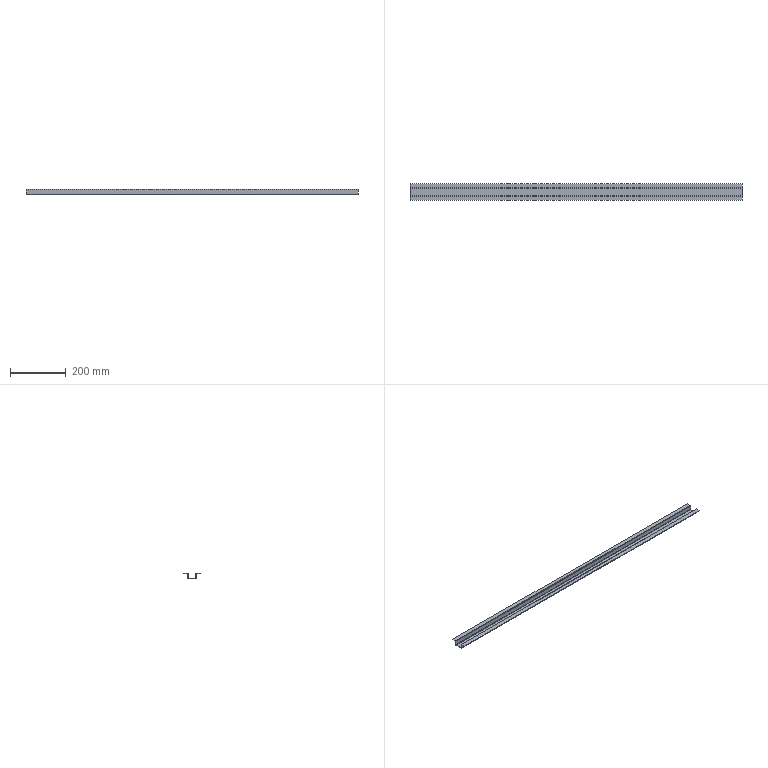Component | SolidWorks | TopPlate-1_TopPanelStiffener-2 | 1 solid | 38 faces | box 1196 x 60 x 18.4 mm | volume 88788 mm3 | plane 30 | cylinder 8 | commonest cylinder face diameters 3.6 x4 2 x4 | material 304
STEP:
#1=COLOUR_RGB('',0.7922,0.8196,0.9333);
#2=FILL_AREA_STYLE_COLOUR('',#1);
#3=FILL_AREA_STYLE('',(#2));
#4=SURFACE_STYLE_FILL_AREA(#3);
#5=SURFACE_SIDE_STYLE('',(#4));
#6=SURFACE_STYLE_USAGE(.BOTH.,#5);
#7=PRESENTATION_STYLE_ASSIGNMENT((#6));
#8=CARTESIAN_POINT('',(-25.908,6.088,79.152));
#9=VERTEX_POINT('',#8);
#10=CARTESIAN_POINT('',(-25.908,6.119,79.152));
#11=VERTEX_POINT('',#10);
#12=CARTESIAN_POINT('',(-25.908,6.088,79.152));
#13=DIRECTION('',(0.,1.,0.));
#14=VECTOR('',#13,39.37);
#15=LINE('',#12,#14);
#16=EDGE_CURVE('',#9,#11,#15,.T.);
#17=ORIENTED_EDGE('',*,*,#16,.F.);
#18=CARTESIAN_POINT('',(-25.908,6.048,79.191));
#19=VERTEX_POINT('',#18);
#20=CARTESIAN_POINT('',(-25.908,6.048,79.152));
#21=DIRECTION('',(1.,-0.,0.));
#22=DIRECTION('',(0.,0.,-1.));
#23=AXIS2_PLACEMENT_3D('',#20,#21,#22);
#24=CIRCLE('',#23,0.03937);
#25=EDGE_CURVE('',#9,#19,#24,.T.);
#26=ORIENTED_EDGE('',*,*,#25,.T.);
#27=CARTESIAN_POINT('',(-25.908,6.048,79.222));
#28=VERTEX_POINT('',#27);
#29=CARTESIAN_POINT('',(-25.908,6.048,79.222));
#30=DIRECTION('',(0.,0.,-1.));
#31=VECTOR('',#30,39.37);
#32=LINE('',#29,#31);
#33=EDGE_CURVE('',#28,#19,#32,.T.);
#34=ORIENTED_EDGE('',*,*,#33,.F.);
#35=CARTESIAN_POINT('',(-25.908,6.048,79.152));
#36=DIRECTION('',(1.,-0.,0.));
#37=DIRECTION('',(0.,1.,0.));
#38=AXIS2_PLACEMENT_3D('',#35,#36,#37);
#39=CIRCLE('',#38,0.07087);
#40=EDGE_CURVE('',#11,#28,#39,.T.);
#41=ORIENTED_EDGE('',*,*,#40,.F.);
#42=EDGE_LOOP('',(#17,#26,#34,#41));
#43=FACE_OUTER_BOUND('',#42,.T.);
#44=CARTESIAN_POINT('',(-25.908,6.088,79.152));
#45=DIRECTION('',(-1.,0.,-0.));
#46=DIRECTION('',(-0.,-0.,1.));
#47=AXIS2_PLACEMENT_3D('',#44,#45,#46);
#48=PLANE('',#47);
#49=ADVANCED_FACE('',(#43),#48,.T.);
#50=CARTESIAN_POINT('',(-25.908,6.088,78.569));
#51=VERTEX_POINT('',#50);
#52=CARTESIAN_POINT('',(-25.908,6.088,79.191));
#53=DIRECTION('',(-0.,-0.,1.));
#54=VECTOR('',#53,39.37);
#55=LINE('',#52,#54);
#56=EDGE_CURVE('',#51,#9,#55,.T.);
#57=ORIENTED_EDGE('',*,*,#56,.T.);
#58=ORIENTED_EDGE('',*,*,#16,.T.);
#59=CARTESIAN_POINT('',(-25.908,6.119,78.569));
#60=VERTEX_POINT('',#59);
#61=CARTESIAN_POINT('',(-25.908,6.119,79.191));
#62=DIRECTION('',(-0.,-0.,1.));
#63=VECTOR('',#62,39.37);
#64=LINE('',#61,#63);
#65=EDGE_CURVE('',#60,#11,#64,.T.);
#66=ORIENTED_EDGE('',*,*,#65,.F.);
#67=CARTESIAN_POINT('',(-25.908,6.119,78.569));
#68=DIRECTION('',(-0.,-1.,-0.));
#69=VECTOR('',#68,39.37);
#70=LINE('',#67,#69);
#71=EDGE_CURVE('',#60,#51,#70,.T.);
#72=ORIENTED_EDGE('',*,*,#71,.T.);
#73=EDGE_LOOP('',(#57,#58,#66,#72));
#74=FACE_OUTER_BOUND('',#73,.T.);
#75=CARTESIAN_POINT('',(-25.908,6.048,79.222));
#76=DIRECTION('',(-1.,0.,-0.));
#77=DIRECTION('',(-0.,-0.,1.));
#78=AXIS2_PLACEMENT_3D('',#75,#76,#77);
#79=PLANE('',#78);
#80=ADVANCED_FACE('',(#74),#79,.T.);
#81=CARTESIAN_POINT('',(21.178,6.048,79.191));
#82=VERTEX_POINT('',#81);
#83=CARTESIAN_POINT('',(21.178,6.048,79.222));
#84=VERTEX_POINT('',#83);
#85=CARTESIAN_POINT('',(21.178,6.048,79.191));
#86=DIRECTION('',(-0.,-0.,1.));
#87=VECTOR('',#86,39.37);
#88=LINE('',#85,#87);
#89=EDGE_CURVE('',#82,#84,#88,.T.);
#90=ORIENTED_EDGE('',*,*,#89,.F.);
#91=CARTESIAN_POINT('',(21.178,6.088,79.152));
#92=VERTEX_POINT('',#91);
#93=CARTESIAN_POINT('',(21.178,6.048,79.152));
#94=DIRECTION('',(1.,-0.,0.));
#95=DIRECTION('',(0.,0.,-1.));
#96=AXIS2_PLACEMENT_3D('',#93,#94,#95);
#97=CIRCLE('',#96,0.03937);
#98=EDGE_CURVE('',#92,#82,#97,.T.);
#99=ORIENTED_EDGE('',*,*,#98,.F.);
#100=CARTESIAN_POINT('',(21.178,6.119,79.152));
#101=VERTEX_POINT('',#100);
#102=CARTESIAN_POINT('',(21.178,6.119,79.152));
#103=DIRECTION('',(-0.,-1.,-0.));
#104=VECTOR('',#103,39.37);
#105=LINE('',#102,#104);
#106=EDGE_CURVE('',#101,#92,#105,.T.);
#107=ORIENTED_EDGE('',*,*,#106,.F.);
#108=CARTESIAN_POINT('',(21.178,6.048,79.152));
#109=DIRECTION('',(1.,-0.,0.));
#110=DIRECTION('',(0.,1.,0.));
#111=AXIS2_PLACEMENT_3D('',#108,#109,#110);
#112=CIRCLE('',#111,0.07087);
#113=EDGE_CURVE('',#101,#84,#112,.T.);
#114=ORIENTED_EDGE('',*,*,#113,.T.);
#115=EDGE_LOOP('',(#90,#99,#107,#114));
#116=FACE_OUTER_BOUND('',#115,.T.);
#117=CARTESIAN_POINT('',(21.178,6.048,79.191));
#118=DIRECTION('',(1.,-0.,0.));
#119=DIRECTION('',(0.,0.,-1.));
#120=AXIS2_PLACEMENT_3D('',#117,#118,#119);
#121=PLANE('',#120);
#122=ADVANCED_FACE('',(#116),#121,.T.);
#123=CARTESIAN_POINT('',(21.178,5.497,79.191));
#124=VERTEX_POINT('',#123);
#125=CARTESIAN_POINT('',(21.178,5.497,79.191));
#126=DIRECTION('',(-0.,-1.,-0.));
#127=VECTOR('',#126,39.37);
#128=LINE('',#125,#127);
#129=EDGE_CURVE('',#82,#124,#128,.T.);
#130=ORIENTED_EDGE('',*,*,#129,.F.);
#131=ORIENTED_EDGE('',*,*,#89,.T.);
#132=CARTESIAN_POINT('',(21.178,5.497,79.222));
#133=VERTEX_POINT('',#132);
#134=CARTESIAN_POINT('',(21.178,5.497,79.222));
#135=DIRECTION('',(-0.,-1.,-0.));
#136=VECTOR('',#135,39.37);
#137=LINE('',#134,#136);
#138=EDGE_CURVE('',#84,#133,#137,.T.);
#139=ORIENTED_EDGE('',*,*,#138,.T.);
#140=CARTESIAN_POINT('',(21.178,5.497,79.222));
#141=DIRECTION('',(0.,0.,-1.));
#142=VECTOR('',#141,39.37);
#143=LINE('',#140,#142);
#144=EDGE_CURVE('',#133,#124,#143,.T.);
#145=ORIENTED_EDGE('',*,*,#144,.T.);
#146=EDGE_LOOP('',(#130,#131,#139,#145));
#147=FACE_OUTER_BOUND('',#146,.T.);
#148=CARTESIAN_POINT('',(21.178,6.119,79.152));
#149=DIRECTION('',(1.,-0.,0.));
#150=DIRECTION('',(0.,0.,-1.));
#151=AXIS2_PLACEMENT_3D('',#148,#149,#150);
#152=PLANE('',#151);
#153=ADVANCED_FACE('',(#147),#152,.T.);
#154=CARTESIAN_POINT('',(-25.908,6.158,78.498));
#155=VERTEX_POINT('',#154);
#156=CARTESIAN_POINT('',(-25.908,6.158,78.53));
#157=VERTEX_POINT('',#156);
#158=CARTESIAN_POINT('',(-25.908,6.158,78.498));
#159=DIRECTION('',(-0.,-0.,1.));
#160=VECTOR('',#159,39.37);
#161=LINE('',#158,#160);
#162=EDGE_CURVE('',#155,#157,#161,.T.);
#163=ORIENTED_EDGE('',*,*,#162,.F.);
#164=CARTESIAN_POINT('',(-25.908,6.158,78.569));
#165=DIRECTION('',(-1.,0.,-0.));
#166=DIRECTION('',(0.,0.,1.));
#167=AXIS2_PLACEMENT_3D('',#164,#165,#166);
#168=CIRCLE('',#167,0.07087);
#169=EDGE_CURVE('',#155,#51,#168,.T.);
#170=ORIENTED_EDGE('',*,*,#169,.T.);
#171=ORIENTED_EDGE('',*,*,#71,.F.);
#172=CARTESIAN_POINT('',(-25.908,6.158,78.569));
#173=DIRECTION('',(-1.,0.,-0.));
#174=DIRECTION('',(0.,1.,0.));
#175=AXIS2_PLACEMENT_3D('',#172,#173,#174);
#176=CIRCLE('',#175,0.03937);
#177=EDGE_CURVE('',#157,#60,#176,.T.);
#178=ORIENTED_EDGE('',*,*,#177,.F.);
#179=EDGE_LOOP('',(#163,#170,#171,#178));
#180=FACE_OUTER_BOUND('',#179,.T.);
#181=CARTESIAN_POINT('',(-25.908,6.158,78.498));
#182=DIRECTION('',(-1.,0.,-0.));
#183=DIRECTION('',(-0.,-0.,1.));
#184=AXIS2_PLACEMENT_3D('',#181,#182,#183);
#185=PLANE('',#184);
#186=ADVANCED_FACE('',(#180),#185,.T.);
#187=CARTESIAN_POINT('',(-25.908,7.198,78.498));
#188=VERTEX_POINT('',#187);
#189=CARTESIAN_POINT('',(-25.908,6.088,78.498));
#190=DIRECTION('',(-0.,-1.,-0.));
#191=VECTOR('',#190,39.37);
#192=LINE('',#189,#191);
#193=EDGE_CURVE('',#188,#155,#192,.T.);
#194=ORIENTED_EDGE('',*,*,#193,.T.);
#195=ORIENTED_EDGE('',*,*,#162,.T.);
#196=CARTESIAN_POINT('',(-25.908,7.198,78.53));
#197=VERTEX_POINT('',#196);
#198=CARTESIAN_POINT('',(-25.908,6.088,78.53));
#199=DIRECTION('',(-0.,-1.,-0.));
#200=VECTOR('',#199,39.37);
#201=LINE('',#198,#200);
#202=EDGE_CURVE('',#197,#157,#201,.T.);
#203=ORIENTED_EDGE('',*,*,#202,.F.);
#204=CARTESIAN_POINT('',(-25.908,7.198,78.53));
#205=DIRECTION('',(0.,0.,-1.));
#206=VECTOR('',#205,39.37);
#207=LINE('',#204,#206);
#208=EDGE_CURVE('',#197,#188,#207,.T.);
#209=ORIENTED_EDGE('',*,*,#208,.T.);
#210=EDGE_LOOP('',(#194,#195,#203,#209));
#211=FACE_OUTER_BOUND('',#210,.T.);
#212=CARTESIAN_POINT('',(-25.908,6.119,78.569));
#213=DIRECTION('',(-1.,0.,-0.));
#214=DIRECTION('',(-0.,-0.,1.));
#215=AXIS2_PLACEMENT_3D('',#212,#213,#214);
#216=PLANE('',#215);
#217=ADVANCED_FACE('',(#211),#216,.T.);
#218=CARTESIAN_POINT('',(21.178,6.088,78.569));
#219=VERTEX_POINT('',#218);
#220=CARTESIAN_POINT('',(21.178,6.119,78.569));
#221=VERTEX_POINT('',#220);
#222=CARTESIAN_POINT('',(21.178,6.088,78.569));
#223=DIRECTION('',(0.,1.,0.));
#224=VECTOR('',#223,39.37);
#225=LINE('',#222,#224);
#226=EDGE_CURVE('',#219,#221,#225,.T.);
#227=ORIENTED_EDGE('',*,*,#226,.F.);
#228=CARTESIAN_POINT('',(21.178,6.158,78.498));
#229=VERTEX_POINT('',#228);
#230=CARTESIAN_POINT('',(21.178,6.158,78.569));
#231=DIRECTION('',(-1.,0.,-0.));
#232=DIRECTION('',(0.,0.,1.));
#233=AXIS2_PLACEMENT_3D('',#230,#231,#232);
#234=CIRCLE('',#233,0.07087);
#235=EDGE_CURVE('',#229,#219,#234,.T.);
#236=ORIENTED_EDGE('',*,*,#235,.F.);
#237=CARTESIAN_POINT('',(21.178,6.158,78.53));
#238=VERTEX_POINT('',#237);
#239=CARTESIAN_POINT('',(21.178,6.158,78.53));
#240=DIRECTION('',(0.,0.,-1.));
#241=VECTOR('',#240,39.37);
#242=LINE('',#239,#241);
#243=EDGE_CURVE('',#238,#229,#242,.T.);
#244=ORIENTED_EDGE('',*,*,#243,.F.);
#245=CARTESIAN_POINT('',(21.178,6.158,78.569));
#246=DIRECTION('',(-1.,0.,-0.));
#247=DIRECTION('',(0.,1.,0.));
#248=AXIS2_PLACEMENT_3D('',#245,#246,#247);
#249=CIRCLE('',#248,0.03937);
#250=EDGE_CURVE('',#238,#221,#249,.T.);
#251=ORIENTED_EDGE('',*,*,#250,.T.);
#252=EDGE_LOOP('',(#227,#236,#244,#251));
#253=FACE_OUTER_BOUND('',#252,.T.);
#254=CARTESIAN_POINT('',(21.178,6.088,78.569));
#255=DIRECTION('',(1.,-0.,0.));
#256=DIRECTION('',(0.,0.,-1.));
#257=AXIS2_PLACEMENT_3D('',#254,#255,#256);
#258=PLANE('',#257);
#259=ADVANCED_FACE('',(#253),#258,.T.);
#260=CARTESIAN_POINT('',(21.178,6.088,79.191));
#261=DIRECTION('',(-0.,-0.,1.));
#262=VECTOR('',#261,39.37);
#263=LINE('',#260,#262);
#264=EDGE_CURVE('',#219,#92,#263,.T.);
#265=ORIENTED_EDGE('',*,*,#264,.F.);
#266=ORIENTED_EDGE('',*,*,#226,.T.);
#267=CARTESIAN_POINT('',(21.178,6.119,79.191));
#268=DIRECTION('',(-0.,-0.,1.));
#269=VECTOR('',#268,39.37);
#270=LINE('',#267,#269);
#271=EDGE_CURVE('',#221,#101,#270,.T.);
#272=ORIENTED_EDGE('',*,*,#271,.T.);
#273=ORIENTED_EDGE('',*,*,#106,.T.);
#274=EDGE_LOOP('',(#265,#266,#272,#273));
#275=FACE_OUTER_BOUND('',#274,.T.);
#276=CARTESIAN_POINT('',(21.178,6.158,78.53));
#277=DIRECTION('',(1.,-0.,0.));
#278=DIRECTION('',(0.,0.,-1.));
#279=AXIS2_PLACEMENT_3D('',#276,#277,#278);
#280=PLANE('',#279);
#281=ADVANCED_FACE('',(#275),#280,.T.);
#282=CARTESIAN_POINT('',(-25.908,7.269,78.569));
#283=VERTEX_POINT('',#282);
#284=CARTESIAN_POINT('',(-25.908,7.237,78.569));
#285=VERTEX_POINT('',#284);
#286=CARTESIAN_POINT('',(-25.908,7.269,78.569));
#287=DIRECTION('',(-0.,-1.,-0.));
#288=VECTOR('',#287,39.37);
#289=LINE('',#286,#288);
#290=EDGE_CURVE('',#283,#285,#289,.T.);
#291=ORIENTED_EDGE('',*,*,#290,.F.);
#292=CARTESIAN_POINT('',(-25.908,7.198,78.569));
#293=DIRECTION('',(-1.,0.,-0.));
#294=DIRECTION('',(0.,0.,1.));
#295=AXIS2_PLACEMENT_3D('',#292,#293,#294);
#296=CIRCLE('',#295,0.07087);
#297=EDGE_CURVE('',#283,#188,#296,.T.);
#298=ORIENTED_EDGE('',*,*,#297,.T.);
#299=ORIENTED_EDGE('',*,*,#208,.F.);
#300=CARTESIAN_POINT('',(-25.908,7.198,78.569));
#301=DIRECTION('',(-1.,0.,-0.));
#302=DIRECTION('',(0.,1.,0.));
#303=AXIS2_PLACEMENT_3D('',#300,#301,#302);
#304=CIRCLE('',#303,0.03937);
#305=EDGE_CURVE('',#285,#197,#304,.T.);
#306=ORIENTED_EDGE('',*,*,#305,.F.);
#307=EDGE_LOOP('',(#291,#298,#299,#306));
#308=FACE_OUTER_BOUND('',#307,.T.);
#309=CARTESIAN_POINT('',(-25.908,7.269,78.569));
#310=DIRECTION('',(-1.,0.,-0.));
#311=DIRECTION('',(-0.,-0.,1.));
#312=AXIS2_PLACEMENT_3D('',#309,#310,#311);
#313=PLANE('',#312);
#314=ADVANCED_FACE('',(#308),#313,.T.);
#315=CARTESIAN_POINT('',(-25.908,7.269,79.152));
#316=VERTEX_POINT('',#315);
#317=CARTESIAN_POINT('',(-25.908,7.269,79.191));
#318=DIRECTION('',(0.,0.,-1.));
#319=VECTOR('',#318,39.37);
#320=LINE('',#317,#319);
#321=EDGE_CURVE('',#316,#283,#320,.T.);
#322=ORIENTED_EDGE('',*,*,#321,.T.);
#323=ORIENTED_EDGE('',*,*,#290,.T.);
#324=CARTESIAN_POINT('',(-25.908,7.237,79.152));
#325=VERTEX_POINT('',#324);
#326=CARTESIAN_POINT('',(-25.908,7.237,79.191));
#327=DIRECTION('',(0.,0.,-1.));
#328=VECTOR('',#327,39.37);
#329=LINE('',#326,#328);
#330=EDGE_CURVE('',#325,#285,#329,.T.);
#331=ORIENTED_EDGE('',*,*,#330,.F.);
#332=CARTESIAN_POINT('',(-25.908,7.237,79.152));
#333=DIRECTION('',(0.,1.,0.));
#334=VECTOR('',#333,39.37);
#335=LINE('',#332,#334);
#336=EDGE_CURVE('',#325,#316,#335,.T.);
#337=ORIENTED_EDGE('',*,*,#336,.T.);
#338=EDGE_LOOP('',(#322,#323,#331,#337));
#339=FACE_OUTER_BOUND('',#338,.T.);
#340=CARTESIAN_POINT('',(-25.908,7.198,78.53));
#341=DIRECTION('',(-1.,0.,-0.));
#342=DIRECTION('',(-0.,-0.,1.));
#343=AXIS2_PLACEMENT_3D('',#340,#341,#342);
#344=PLANE('',#343);
#345=ADVANCED_FACE('',(#339),#344,.T.);
#346=CARTESIAN_POINT('',(21.178,7.198,78.498));
#347=VERTEX_POINT('',#346);
#348=CARTESIAN_POINT('',(21.178,7.198,78.53));
#349=VERTEX_POINT('',#348);
#350=CARTESIAN_POINT('',(21.178,7.198,78.498));
#351=DIRECTION('',(-0.,-0.,1.));
#352=VECTOR('',#351,39.37);
#353=LINE('',#350,#352);
#354=EDGE_CURVE('',#347,#349,#353,.T.);
#355=ORIENTED_EDGE('',*,*,#354,.F.);
#356=CARTESIAN_POINT('',(21.178,7.269,78.569));
#357=VERTEX_POINT('',#356);
#358=CARTESIAN_POINT('',(21.178,7.198,78.569));
#359=DIRECTION('',(-1.,0.,-0.));
#360=DIRECTION('',(0.,0.,1.));
#361=AXIS2_PLACEMENT_3D('',#358,#359,#360);
#362=CIRCLE('',#361,0.07087);
#363=EDGE_CURVE('',#357,#347,#362,.T.);
#364=ORIENTED_EDGE('',*,*,#363,.F.);
#365=CARTESIAN_POINT('',(21.178,7.237,78.569));
#366=VERTEX_POINT('',#365);
#367=CARTESIAN_POINT('',(21.178,7.237,78.569));
#368=DIRECTION('',(0.,1.,0.));
#369=VECTOR('',#368,39.37);
#370=LINE('',#367,#369);
#371=EDGE_CURVE('',#366,#357,#370,.T.);
#372=ORIENTED_EDGE('',*,*,#371,.F.);
#373=CARTESIAN_POINT('',(21.178,7.198,78.569));
#374=DIRECTION('',(-1.,0.,-0.));
#375=DIRECTION('',(0.,1.,0.));
#376=AXIS2_PLACEMENT_3D('',#373,#374,#375);
#377=CIRCLE('',#376,0.03937);
#378=EDGE_CURVE('',#366,#349,#377,.T.);
#379=ORIENTED_EDGE('',*,*,#378,.T.);
#380=EDGE_LOOP('',(#355,#364,#372,#379));
#381=FACE_OUTER_BOUND('',#380,.T.);
#382=CARTESIAN_POINT('',(21.178,7.198,78.498));
#383=DIRECTION('',(1.,-0.,0.));
#384=DIRECTION('',(0.,0.,-1.));
#385=AXIS2_PLACEMENT_3D('',#382,#383,#384);
#386=PLANE('',#385);
#387=ADVANCED_FACE('',(#381),#386,.T.);
#388=CARTESIAN_POINT('',(21.178,6.088,78.498));
#389=DIRECTION('',(-0.,-1.,-0.));
#390=VECTOR('',#389,39.37);
#391=LINE('',#388,#390);
#392=EDGE_CURVE('',#347,#229,#391,.T.);
#393=ORIENTED_EDGE('',*,*,#392,.F.);
#394=ORIENTED_EDGE('',*,*,#354,.T.);
#395=CARTESIAN_POINT('',(21.178,6.088,78.53));
#396=DIRECTION('',(-0.,-1.,-0.));
#397=VECTOR('',#396,39.37);
#398=LINE('',#395,#397);
#399=EDGE_CURVE('',#349,#238,#398,.T.);
#400=ORIENTED_EDGE('',*,*,#399,.T.);
#401=ORIENTED_EDGE('',*,*,#243,.T.);
#402=EDGE_LOOP('',(#393,#394,#400,#401));
#403=FACE_OUTER_BOUND('',#402,.T.);
#404=CARTESIAN_POINT('',(21.178,7.237,78.569));
#405=DIRECTION('',(1.,-0.,0.));
#406=DIRECTION('',(0.,0.,-1.));
#407=AXIS2_PLACEMENT_3D('',#404,#405,#406);
#408=PLANE('',#407);
#409=ADVANCED_FACE('',(#403),#408,.T.);
#410=CARTESIAN_POINT('',(-25.908,7.308,79.191));
#411=VERTEX_POINT('',#410);
#412=CARTESIAN_POINT('',(-25.908,7.308,79.222));
#413=VERTEX_POINT('',#412);
#414=CARTESIAN_POINT('',(-25.908,7.308,79.191));
#415=DIRECTION('',(-0.,-0.,1.));
#416=VECTOR('',#415,39.37);
#417=LINE('',#414,#416);
#418=EDGE_CURVE('',#411,#413,#417,.T.);
#419=ORIENTED_EDGE('',*,*,#418,.F.);
#420=CARTESIAN_POINT('',(-25.908,7.308,79.152));
#421=DIRECTION('',(1.,-0.,0.));
#422=DIRECTION('',(0.,0.,-1.));
#423=AXIS2_PLACEMENT_3D('',#420,#421,#422);
#424=CIRCLE('',#423,0.03937);
#425=EDGE_CURVE('',#411,#316,#424,.T.);
#426=ORIENTED_EDGE('',*,*,#425,.T.);
#427=ORIENTED_EDGE('',*,*,#336,.F.);
#428=CARTESIAN_POINT('',(-25.908,7.308,79.152));
#429=DIRECTION('',(1.,-0.,0.));
#430=DIRECTION('',(0.,1.,0.));
#431=AXIS2_PLACEMENT_3D('',#428,#429,#430);
#432=CIRCLE('',#431,0.07087);
#433=EDGE_CURVE('',#413,#325,#432,.T.);
#434=ORIENTED_EDGE('',*,*,#433,.F.);
#435=EDGE_LOOP('',(#419,#426,#427,#434));
#436=FACE_OUTER_BOUND('',#435,.T.);
#437=CARTESIAN_POINT('',(-25.908,7.308,79.191));
#438=DIRECTION('',(-1.,0.,-0.));
#439=DIRECTION('',(-0.,-0.,1.));
#440=AXIS2_PLACEMENT_3D('',#437,#438,#439);
#441=PLANE('',#440);
#442=ADVANCED_FACE('',(#436),#441,.T.);
#443=CARTESIAN_POINT('',(-25.908,7.859,79.191));
#444=VERTEX_POINT('',#443);
#445=CARTESIAN_POINT('',(-25.908,7.859,79.191));
#446=DIRECTION('',(-0.,-1.,-0.));
#447=VECTOR('',#446,39.37);
#448=LINE('',#445,#447);
#449=EDGE_CURVE('',#444,#411,#448,.T.);
#450=ORIENTED_EDGE('',*,*,#449,.T.);
#451=ORIENTED_EDGE('',*,*,#418,.T.);
#452=CARTESIAN_POINT('',(-25.908,7.859,79.222));
#453=VERTEX_POINT('',#452);
#454=CARTESIAN_POINT('',(-25.908,7.859,79.222));
#455=DIRECTION('',(-0.,-1.,-0.));
#456=VECTOR('',#455,39.37);
#457=LINE('',#454,#456);
#458=EDGE_CURVE('',#453,#413,#457,.T.);
#459=ORIENTED_EDGE('',*,*,#458,.F.);
#460=CARTESIAN_POINT('',(-25.908,7.859,79.191));
#461=DIRECTION('',(-0.,-0.,1.));
#462=VECTOR('',#461,39.37);
#463=LINE('',#460,#462);
#464=EDGE_CURVE('',#444,#453,#463,.T.);
#465=ORIENTED_EDGE('',*,*,#464,.F.);
#466=EDGE_LOOP('',(#450,#451,#459,#465));
#467=FACE_OUTER_BOUND('',#466,.T.);
#468=CARTESIAN_POINT('',(-25.908,7.237,79.152));
#469=DIRECTION('',(-1.,0.,-0.));
#470=DIRECTION('',(-0.,-0.,1.));
#471=AXIS2_PLACEMENT_3D('',#468,#469,#470);
#472=PLANE('',#471);
#473=ADVANCED_FACE('',(#467),#472,.T.);
#474=CARTESIAN_POINT('',(21.178,7.269,79.152));
#475=VERTEX_POINT('',#474);
#476=CARTESIAN_POINT('',(21.178,7.237,79.152));
#477=VERTEX_POINT('',#476);
#478=CARTESIAN_POINT('',(21.178,7.269,79.152));
#479=DIRECTION('',(-0.,-1.,-0.));
#480=VECTOR('',#479,39.37);
#481=LINE('',#478,#480);
#482=EDGE_CURVE('',#475,#477,#481,.T.);
#483=ORIENTED_EDGE('',*,*,#482,.F.);
#484=CARTESIAN_POINT('',(21.178,7.308,79.191));
#485=VERTEX_POINT('',#484);
#486=CARTESIAN_POINT('',(21.178,7.308,79.152));
#487=DIRECTION('',(1.,-0.,0.));
#488=DIRECTION('',(0.,0.,-1.));
#489=AXIS2_PLACEMENT_3D('',#486,#487,#488);
#490=CIRCLE('',#489,0.03937);
#491=EDGE_CURVE('',#485,#475,#490,.T.);
#492=ORIENTED_EDGE('',*,*,#491,.F.);
#493=CARTESIAN_POINT('',(21.178,7.308,79.222));
#494=VERTEX_POINT('',#493);
#495=CARTESIAN_POINT('',(21.178,7.308,79.222));
#496=DIRECTION('',(0.,0.,-1.));
#497=VECTOR('',#496,39.37);
#498=LINE('',#495,#497);
#499=EDGE_CURVE('',#494,#485,#498,.T.);
#500=ORIENTED_EDGE('',*,*,#499,.F.);
#501=CARTESIAN_POINT('',(21.178,7.308,79.152));
#502=DIRECTION('',(1.,-0.,0.));
#503=DIRECTION('',(0.,1.,0.));
#504=AXIS2_PLACEMENT_3D('',#501,#502,#503);
#505=CIRCLE('',#504,0.07087);
#506=EDGE_CURVE('',#494,#477,#505,.T.);
#507=ORIENTED_EDGE('',*,*,#506,.T.);
#508=EDGE_LOOP('',(#483,#492,#500,#507));
#509=FACE_OUTER_BOUND('',#508,.T.);
#510=CARTESIAN_POINT('',(21.178,7.269,79.152));
#511=DIRECTION('',(1.,-0.,0.));
#512=DIRECTION('',(0.,0.,-1.));
#513=AXIS2_PLACEMENT_3D('',#510,#511,#512);
#514=PLANE('',#513);
#515=ADVANCED_FACE('',(#509),#514,.T.);
#516=CARTESIAN_POINT('',(21.178,7.269,79.191));
#517=DIRECTION('',(0.,0.,-1.));
#518=VECTOR('',#517,39.37);
#519=LINE('',#516,#518);
#520=EDGE_CURVE('',#475,#357,#519,.T.);
#521=ORIENTED_EDGE('',*,*,#520,.F.);
#522=ORIENTED_EDGE('',*,*,#482,.T.);
#523=CARTESIAN_POINT('',(21.178,7.237,79.191));
#524=DIRECTION('',(0.,0.,-1.));
#525=VECTOR('',#524,39.37);
#526=LINE('',#523,#525);
#527=EDGE_CURVE('',#477,#366,#526,.T.);
#528=ORIENTED_EDGE('',*,*,#527,.T.);
#529=ORIENTED_EDGE('',*,*,#371,.T.);
#530=EDGE_LOOP('',(#521,#522,#528,#529));
#531=FACE_OUTER_BOUND('',#530,.T.);
#532=CARTESIAN_POINT('',(21.178,7.308,79.222));
#533=DIRECTION('',(1.,-0.,0.));
#534=DIRECTION('',(0.,0.,-1.));
#535=AXIS2_PLACEMENT_3D('',#532,#533,#534);
#536=PLANE('',#535);
#537=ADVANCED_FACE('',(#531),#536,.T.);
#538=ORIENTED_EDGE('',*,*,#129,.T.);
#539=CARTESIAN_POINT('',(-25.908,5.497,79.191));
#540=VERTEX_POINT('',#539);
#541=CARTESIAN_POINT('',(-25.908,5.497,79.191));
#542=DIRECTION('',(1.,-0.,0.));
#543=VECTOR('',#542,39.37);
#544=LINE('',#541,#543);
#545=EDGE_CURVE('',#540,#124,#544,.T.);
#546=ORIENTED_EDGE('',*,*,#545,.F.);
#547=CARTESIAN_POINT('',(-25.908,5.497,79.191));
#548=DIRECTION('',(-0.,-1.,-0.));
#549=VECTOR('',#548,39.37);
#550=LINE('',#547,#549);
#551=EDGE_CURVE('',#19,#540,#550,.T.);
#552=ORIENTED_EDGE('',*,*,#551,.F.);
#553=CARTESIAN_POINT('',(-25.908,6.048,79.191));
#554=DIRECTION('',(1.,-0.,0.));
#555=VECTOR('',#554,39.37);
#556=LINE('',#553,#555);
#557=EDGE_CURVE('',#19,#82,#556,.T.);
#558=ORIENTED_EDGE('',*,*,#557,.T.);
#559=EDGE_LOOP('',(#538,#546,#552,#558));
#560=FACE_OUTER_BOUND('',#559,.T.);
#561=CARTESIAN_POINT('',(-25.908,5.497,79.191));
#562=DIRECTION('',(-0.,-0.,1.));
#563=DIRECTION('',(0.,1.,0.));
#564=AXIS2_PLACEMENT_3D('',#561,#562,#563);
#565=PLANE('',#564);
#566=ADVANCED_FACE('',(#560),#565,.F.);
#567=ORIENTED_EDGE('',*,*,#144,.F.);
#568=CARTESIAN_POINT('',(-25.908,5.497,79.222));
#569=VERTEX_POINT('',#568);
#570=CARTESIAN_POINT('',(-25.908,5.497,79.222));
#571=DIRECTION('',(1.,-0.,0.));
#572=VECTOR('',#571,39.37);
#573=LINE('',#570,#572);
#574=EDGE_CURVE('',#569,#133,#573,.T.);
#575=ORIENTED_EDGE('',*,*,#574,.F.);
#576=CARTESIAN_POINT('',(-25.908,5.497,79.222));
#577=DIRECTION('',(0.,0.,-1.));
#578=VECTOR('',#577,39.37);
#579=LINE('',#576,#578);
#580=EDGE_CURVE('',#569,#540,#579,.T.);
#581=ORIENTED_EDGE('',*,*,#580,.T.);
#582=ORIENTED_EDGE('',*,*,#545,.T.);
#583=EDGE_LOOP('',(#567,#575,#581,#582));
#584=FACE_OUTER_BOUND('',#583,.T.);
#585=CARTESIAN_POINT('',(-25.908,5.497,79.222));
#586=DIRECTION('',(-0.,-1.,-0.));
#587=DIRECTION('',(-0.,-0.,1.));
#588=AXIS2_PLACEMENT_3D('',#585,#586,#587);
#589=PLANE('',#588);
#590=ADVANCED_FACE('',(#584),#589,.T.);
#591=ORIENTED_EDGE('',*,*,#138,.F.);
#592=CARTESIAN_POINT('',(-25.908,6.048,79.222));
#593=DIRECTION('',(1.,-0.,0.));
#594=VECTOR('',#593,39.37);
#595=LINE('',#592,#594);
#596=EDGE_CURVE('',#28,#84,#595,.T.);
#597=ORIENTED_EDGE('',*,*,#596,.F.);
#598=CARTESIAN_POINT('',(-25.908,5.497,79.222));
#599=DIRECTION('',(-0.,-1.,-0.));
#600=VECTOR('',#599,39.37);
#601=LINE('',#598,#600);
#602=EDGE_CURVE('',#28,#569,#601,.T.);
#603=ORIENTED_EDGE('',*,*,#602,.T.);
#604=ORIENTED_EDGE('',*,*,#574,.T.);
#605=EDGE_LOOP('',(#591,#597,#603,#604));
#606=FACE_OUTER_BOUND('',#605,.T.);
#607=CARTESIAN_POINT('',(-25.908,5.497,79.222));
#608=DIRECTION('',(-0.,-0.,1.));
#609=DIRECTION('',(0.,1.,0.));
#610=AXIS2_PLACEMENT_3D('',#607,#608,#609);
#611=PLANE('',#610);
#612=ADVANCED_FACE('',(#606),#611,.T.);
#613=ORIENTED_EDGE('',*,*,#113,.F.);
#614=CARTESIAN_POINT('',(-25.908,6.119,79.152));
#615=DIRECTION('',(1.,-0.,0.));
#616=VECTOR('',#615,39.37);
#617=LINE('',#614,#616);
#618=EDGE_CURVE('',#11,#101,#617,.T.);
#619=ORIENTED_EDGE('',*,*,#618,.F.);
#620=ORIENTED_EDGE('',*,*,#40,.T.);
#621=ORIENTED_EDGE('',*,*,#596,.T.);
#622=EDGE_LOOP('',(#613,#619,#620,#621));
#623=FACE_OUTER_BOUND('',#622,.T.);
#624=CARTESIAN_POINT('',(-25.908,6.048,79.152));
#625=DIRECTION('',(1.,-0.,0.));
#626=DIRECTION('',(0.,0.,-1.));
#627=AXIS2_PLACEMENT_3D('',#624,#625,#626);
#628=CYLINDRICAL_SURFACE('',#627,0.07087);
#629=ADVANCED_FACE('',(#623),#628,.T.);
#630=ORIENTED_EDGE('',*,*,#271,.F.);
#631=CARTESIAN_POINT('',(-25.908,6.119,78.569));
#632=DIRECTION('',(1.,-0.,0.));
#633=VECTOR('',#632,39.37);
#634=LINE('',#631,#633);
#635=EDGE_CURVE('',#60,#221,#634,.T.);
#636=ORIENTED_EDGE('',*,*,#635,.F.);
#637=ORIENTED_EDGE('',*,*,#65,.T.);
#638=ORIENTED_EDGE('',*,*,#618,.T.);
#639=EDGE_LOOP('',(#630,#636,#637,#638));
#640=FACE_OUTER_BOUND('',#639,.T.);
#641=CARTESIAN_POINT('',(-25.908,6.119,79.191));
#642=DIRECTION('',(0.,1.,0.));
#643=DIRECTION('',(0.,0.,-1.));
#644=AXIS2_PLACEMENT_3D('',#641,#642,#643);
#645=PLANE('',#644);
#646=ADVANCED_FACE('',(#640),#645,.T.);
#647=ORIENTED_EDGE('',*,*,#250,.F.);
#648=CARTESIAN_POINT('',(-25.908,6.158,78.53));
#649=DIRECTION('',(1.,-0.,0.));
#650=VECTOR('',#649,39.37);
#651=LINE('',#648,#650);
#652=EDGE_CURVE('',#157,#238,#651,.T.);
#653=ORIENTED_EDGE('',*,*,#652,.F.);
#654=ORIENTED_EDGE('',*,*,#177,.T.);
#655=ORIENTED_EDGE('',*,*,#635,.T.);
#656=EDGE_LOOP('',(#647,#653,#654,#655));
#657=FACE_OUTER_BOUND('',#656,.T.);
#658=CARTESIAN_POINT('',(-25.908,6.158,78.569));
#659=DIRECTION('',(1.,-0.,0.));
#660=DIRECTION('',(0.,0.,-1.));
#661=AXIS2_PLACEMENT_3D('',#658,#659,#660);
#662=CYLINDRICAL_SURFACE('',#661,0.03937);
#663=ADVANCED_FACE('',(#657),#662,.F.);
#664=ORIENTED_EDGE('',*,*,#399,.F.);
#665=CARTESIAN_POINT('',(-25.908,7.198,78.53));
#666=DIRECTION('',(1.,-0.,0.));
#667=VECTOR('',#666,39.37);
#668=LINE('',#665,#667);
#669=EDGE_CURVE('',#197,#349,#668,.T.);
#670=ORIENTED_EDGE('',*,*,#669,.F.);
#671=ORIENTED_EDGE('',*,*,#202,.T.);
#672=ORIENTED_EDGE('',*,*,#652,.T.);
#673=EDGE_LOOP('',(#664,#670,#671,#672));
#674=FACE_OUTER_BOUND('',#673,.T.);
#675=CARTESIAN_POINT('',(-25.908,6.088,78.53));
#676=DIRECTION('',(-0.,-0.,1.));
#677=DIRECTION('',(0.,1.,0.));
#678=AXIS2_PLACEMENT_3D('',#675,#676,#677);
#679=PLANE('',#678);
#680=ADVANCED_FACE('',(#674),#679,.T.);
#681=ORIENTED_EDGE('',*,*,#378,.F.);
#682=CARTESIAN_POINT('',(-25.908,7.237,78.569));
#683=DIRECTION('',(1.,-0.,0.));
#684=VECTOR('',#683,39.37);
#685=LINE('',#682,#684);
#686=EDGE_CURVE('',#285,#366,#685,.T.);
#687=ORIENTED_EDGE('',*,*,#686,.F.);
#688=ORIENTED_EDGE('',*,*,#305,.T.);
#689=ORIENTED_EDGE('',*,*,#669,.T.);
#690=EDGE_LOOP('',(#681,#687,#688,#689));
#691=FACE_OUTER_BOUND('',#690,.T.);
#692=CARTESIAN_POINT('',(-25.908,7.198,78.569));
#693=DIRECTION('',(1.,-0.,0.));
#694=DIRECTION('',(0.,0.,-1.));
#695=AXIS2_PLACEMENT_3D('',#692,#693,#694);
#696=CYLINDRICAL_SURFACE('',#695,0.03937);
#697=ADVANCED_FACE('',(#691),#696,.F.);
#698=ORIENTED_EDGE('',*,*,#527,.F.);
#699=CARTESIAN_POINT('',(-25.908,7.237,79.152));
#700=DIRECTION('',(1.,-0.,0.));
#701=VECTOR('',#700,39.37);
#702=LINE('',#699,#701);
#703=EDGE_CURVE('',#325,#477,#702,.T.);
#704=ORIENTED_EDGE('',*,*,#703,.F.);
#705=ORIENTED_EDGE('',*,*,#330,.T.);
#706=ORIENTED_EDGE('',*,*,#686,.T.);
#707=EDGE_LOOP('',(#698,#704,#705,#706));
#708=FACE_OUTER_BOUND('',#707,.T.);
#709=CARTESIAN_POINT('',(-25.908,7.237,79.191));
#710=DIRECTION('',(-0.,-1.,-0.));
#711=DIRECTION('',(-0.,-0.,1.));
#712=AXIS2_PLACEMENT_3D('',#709,#710,#711);
#713=PLANE('',#712);
#714=ADVANCED_FACE('',(#708),#713,.T.);
#715=ORIENTED_EDGE('',*,*,#506,.F.);
#716=CARTESIAN_POINT('',(-25.908,7.308,79.222));
#717=DIRECTION('',(1.,-0.,0.));
#718=VECTOR('',#717,39.37);
#719=LINE('',#716,#718);
#720=EDGE_CURVE('',#413,#494,#719,.T.);
#721=ORIENTED_EDGE('',*,*,#720,.F.);
#722=ORIENTED_EDGE('',*,*,#433,.T.);
#723=ORIENTED_EDGE('',*,*,#703,.T.);
#724=EDGE_LOOP('',(#715,#721,#722,#723));
#725=FACE_OUTER_BOUND('',#724,.T.);
#726=CARTESIAN_POINT('',(-25.908,7.308,79.152));
#727=DIRECTION('',(1.,-0.,0.));
#728=DIRECTION('',(0.,0.,-1.));
#729=AXIS2_PLACEMENT_3D('',#726,#727,#728);
#730=CYLINDRICAL_SURFACE('',#729,0.07087);
#731=ADVANCED_FACE('',(#725),#730,.T.);
#732=CARTESIAN_POINT('',(21.178,7.859,79.222));
#733=VERTEX_POINT('',#732);
#734=CARTESIAN_POINT('',(21.178,7.859,79.222));
#735=DIRECTION('',(-0.,-1.,-0.));
#736=VECTOR('',#735,39.37);
#737=LINE('',#734,#736);
#738=EDGE_CURVE('',#733,#494,#737,.T.);
#739=ORIENTED_EDGE('',*,*,#738,.F.);
#740=CARTESIAN_POINT('',(-25.908,7.859,79.222));
#741=DIRECTION('',(1.,-0.,0.));
#742=VECTOR('',#741,39.37);
#743=LINE('',#740,#742);
#744=EDGE_CURVE('',#453,#733,#743,.T.);
#745=ORIENTED_EDGE('',*,*,#744,.F.);
#746=ORIENTED_EDGE('',*,*,#458,.T.);
#747=ORIENTED_EDGE('',*,*,#720,.T.);
#748=EDGE_LOOP('',(#739,#745,#746,#747));
#749=FACE_OUTER_BOUND('',#748,.T.);
#750=CARTESIAN_POINT('',(-25.908,7.859,79.222));
#751=DIRECTION('',(-0.,-0.,1.));
#752=DIRECTION('',(0.,1.,0.));
#753=AXIS2_PLACEMENT_3D('',#750,#751,#752);
#754=PLANE('',#753);
#755=ADVANCED_FACE('',(#749),#754,.T.);
#756=CARTESIAN_POINT('',(21.178,7.859,79.191));
#757=VERTEX_POINT('',#756);
#758=CARTESIAN_POINT('',(21.178,7.859,79.191));
#759=DIRECTION('',(-0.,-0.,1.));
#760=VECTOR('',#759,39.37);
#761=LINE('',#758,#760);
#762=EDGE_CURVE('',#757,#733,#761,.T.);
#763=ORIENTED_EDGE('',*,*,#762,.F.);
#764=CARTESIAN_POINT('',(-25.908,7.859,79.191));
#765=DIRECTION('',(1.,-0.,0.));
#766=VECTOR('',#765,39.37);
#767=LINE('',#764,#766);
#768=EDGE_CURVE('',#444,#757,#767,.T.);
#769=ORIENTED_EDGE('',*,*,#768,.F.);
#770=ORIENTED_EDGE('',*,*,#464,.T.);
#771=ORIENTED_EDGE('',*,*,#744,.T.);
#772=EDGE_LOOP('',(#763,#769,#770,#771));
#773=FACE_OUTER_BOUND('',#772,.T.);
#774=CARTESIAN_POINT('',(-25.908,7.859,79.191));
#775=DIRECTION('',(0.,1.,0.));
#776=DIRECTION('',(0.,0.,-1.));
#777=AXIS2_PLACEMENT_3D('',#774,#775,#776);
#778=PLANE('',#777);
#779=ADVANCED_FACE('',(#773),#778,.T.);
#780=CARTESIAN_POINT('',(21.178,7.859,79.191));
#781=DIRECTION('',(-0.,-1.,-0.));
#782=VECTOR('',#781,39.37);
#783=LINE('',#780,#782);
#784=EDGE_CURVE('',#757,#485,#783,.T.);
#785=ORIENTED_EDGE('',*,*,#784,.T.);
#786=CARTESIAN_POINT('',(-25.908,7.308,79.191));
#787=DIRECTION('',(1.,-0.,0.));
#788=VECTOR('',#787,39.37);
#789=LINE('',#786,#788);
#790=EDGE_CURVE('',#411,#485,#789,.T.);
#791=ORIENTED_EDGE('',*,*,#790,.F.);
#792=ORIENTED_EDGE('',*,*,#449,.F.);
#793=ORIENTED_EDGE('',*,*,#768,.T.);
#794=EDGE_LOOP('',(#785,#791,#792,#793));
#795=FACE_OUTER_BOUND('',#794,.T.);
#796=CARTESIAN_POINT('',(-25.908,7.859,79.191));
#797=DIRECTION('',(-0.,-0.,1.));
#798=DIRECTION('',(0.,1.,0.));
#799=AXIS2_PLACEMENT_3D('',#796,#797,#798);
#800=PLANE('',#799);
#801=ADVANCED_FACE('',(#795),#800,.F.);
#802=ORIENTED_EDGE('',*,*,#491,.T.);
#803=CARTESIAN_POINT('',(-25.908,7.269,79.152));
#804=DIRECTION('',(1.,-0.,0.));
#805=VECTOR('',#804,39.37);
#806=LINE('',#803,#805);
#807=EDGE_CURVE('',#316,#475,#806,.T.);
#808=ORIENTED_EDGE('',*,*,#807,.F.);
#809=ORIENTED_EDGE('',*,*,#425,.F.);
#810=ORIENTED_EDGE('',*,*,#790,.T.);
#811=EDGE_LOOP('',(#802,#808,#809,#810));
#812=FACE_OUTER_BOUND('',#811,.T.);
#813=CARTESIAN_POINT('',(-25.908,7.308,79.152));
#814=DIRECTION('',(1.,-0.,0.));
#815=DIRECTION('',(0.,0.,-1.));
#816=AXIS2_PLACEMENT_3D('',#813,#814,#815);
#817=CYLINDRICAL_SURFACE('',#816,0.03937);
#818=ADVANCED_FACE('',(#812),#817,.F.);
#819=ORIENTED_EDGE('',*,*,#520,.T.);
#820=CARTESIAN_POINT('',(-25.908,7.269,78.569));
#821=DIRECTION('',(1.,-0.,0.));
#822=VECTOR('',#821,39.37);
#823=LINE('',#820,#822);
#824=EDGE_CURVE('',#283,#357,#823,.T.);
#825=ORIENTED_EDGE('',*,*,#824,.F.);
#826=ORIENTED_EDGE('',*,*,#321,.F.);
#827=ORIENTED_EDGE('',*,*,#807,.T.);
#828=EDGE_LOOP('',(#819,#825,#826,#827));
#829=FACE_OUTER_BOUND('',#828,.T.);
#830=CARTESIAN_POINT('',(-25.908,7.269,79.191));
#831=DIRECTION('',(-0.,-1.,-0.));
#832=DIRECTION('',(-0.,-0.,1.));
#833=AXIS2_PLACEMENT_3D('',#830,#831,#832);
#834=PLANE('',#833);
#835=ADVANCED_FACE('',(#829),#834,.F.);
#836=ORIENTED_EDGE('',*,*,#363,.T.);
#837=CARTESIAN_POINT('',(-25.908,7.198,78.498));
#838=DIRECTION('',(1.,-0.,0.));
#839=VECTOR('',#838,39.37);
#840=LINE('',#837,#839);
#841=EDGE_CURVE('',#188,#347,#840,.T.);
#842=ORIENTED_EDGE('',*,*,#841,.F.);
#843=ORIENTED_EDGE('',*,*,#297,.F.);
#844=ORIENTED_EDGE('',*,*,#824,.T.);
#845=EDGE_LOOP('',(#836,#842,#843,#844));
#846=FACE_OUTER_BOUND('',#845,.T.);
#847=CARTESIAN_POINT('',(-25.908,7.198,78.569));
#848=DIRECTION('',(1.,-0.,0.));
#849=DIRECTION('',(0.,0.,-1.));
#850=AXIS2_PLACEMENT_3D('',#847,#848,#849);
#851=CYLINDRICAL_SURFACE('',#850,0.07087);
#852=ADVANCED_FACE('',(#846),#851,.T.);
#853=ORIENTED_EDGE('',*,*,#392,.T.);
#854=CARTESIAN_POINT('',(-25.908,6.158,78.498));
#855=DIRECTION('',(1.,-0.,0.));
#856=VECTOR('',#855,39.37);
#857=LINE('',#854,#856);
#858=EDGE_CURVE('',#155,#229,#857,.T.);
#859=ORIENTED_EDGE('',*,*,#858,.F.);
#860=ORIENTED_EDGE('',*,*,#193,.F.);
#861=ORIENTED_EDGE('',*,*,#841,.T.);
#862=EDGE_LOOP('',(#853,#859,#860,#861));
#863=FACE_OUTER_BOUND('',#862,.T.);
#864=CARTESIAN_POINT('',(-25.908,6.088,78.498));
#865=DIRECTION('',(-0.,-0.,1.));
#866=DIRECTION('',(0.,1.,0.));
#867=AXIS2_PLACEMENT_3D('',#864,#865,#866);
#868=PLANE('',#867);
#869=ADVANCED_FACE('',(#863),#868,.F.);
#870=ORIENTED_EDGE('',*,*,#235,.T.);
#871=CARTESIAN_POINT('',(-25.908,6.088,78.569));
#872=DIRECTION('',(1.,-0.,0.));
#873=VECTOR('',#872,39.37);
#874=LINE('',#871,#873);
#875=EDGE_CURVE('',#51,#219,#874,.T.);
#876=ORIENTED_EDGE('',*,*,#875,.F.);
#877=ORIENTED_EDGE('',*,*,#169,.F.);
#878=ORIENTED_EDGE('',*,*,#858,.T.);
#879=EDGE_LOOP('',(#870,#876,#877,#878));
#880=FACE_OUTER_BOUND('',#879,.T.);
#881=CARTESIAN_POINT('',(-25.908,6.158,78.569));
#882=DIRECTION('',(1.,-0.,0.));
#883=DIRECTION('',(0.,0.,-1.));
#884=AXIS2_PLACEMENT_3D('',#881,#882,#883);
#885=CYLINDRICAL_SURFACE('',#884,0.07087);
#886=ADVANCED_FACE('',(#880),#885,.T.);
#887=ORIENTED_EDGE('',*,*,#264,.T.);
#888=CARTESIAN_POINT('',(-25.908,6.088,79.152));
#889=DIRECTION('',(1.,-0.,0.));
#890=VECTOR('',#889,39.37);
#891=LINE('',#888,#890);
#892=EDGE_CURVE('',#9,#92,#891,.T.);
#893=ORIENTED_EDGE('',*,*,#892,.F.);
#894=ORIENTED_EDGE('',*,*,#56,.F.);
#895=ORIENTED_EDGE('',*,*,#875,.T.);
#896=EDGE_LOOP('',(#887,#893,#894,#895));
#897=FACE_OUTER_BOUND('',#896,.T.);
#898=CARTESIAN_POINT('',(-25.908,6.088,79.191));
#899=DIRECTION('',(0.,1.,0.));
#900=DIRECTION('',(0.,0.,-1.));
#901=AXIS2_PLACEMENT_3D('',#898,#899,#900);
#902=PLANE('',#901);
#903=ADVANCED_FACE('',(#897),#902,.F.);
#904=ORIENTED_EDGE('',*,*,#98,.T.);
#905=ORIENTED_EDGE('',*,*,#557,.F.);
#906=ORIENTED_EDGE('',*,*,#25,.F.);
#907=ORIENTED_EDGE('',*,*,#892,.T.);
#908=EDGE_LOOP('',(#904,#905,#906,#907));
#909=FACE_OUTER_BOUND('',#908,.T.);
#910=CARTESIAN_POINT('',(-25.908,6.048,79.152));
#911=DIRECTION('',(1.,-0.,0.));
#912=DIRECTION('',(0.,0.,-1.));
#913=AXIS2_PLACEMENT_3D('',#910,#911,#912);
#914=CYLINDRICAL_SURFACE('',#913,0.03937);
#915=ADVANCED_FACE('',(#909),#914,.F.);
#916=ORIENTED_EDGE('',*,*,#551,.T.);
#917=ORIENTED_EDGE('',*,*,#580,.F.);
#918=ORIENTED_EDGE('',*,*,#602,.F.);
#919=ORIENTED_EDGE('',*,*,#33,.T.);
#920=EDGE_LOOP('',(#916,#917,#918,#919));
#921=FACE_OUTER_BOUND('',#920,.T.);
#922=CARTESIAN_POINT('',(-25.908,6.048,79.152));
#923=DIRECTION('',(-1.,0.,-0.));
#924=DIRECTION('',(0.,1.,0.));
#925=AXIS2_PLACEMENT_3D('',#922,#923,#924);
#926=PLANE('',#925);
#927=ADVANCED_FACE('',(#921),#926,.T.);
#928=ORIENTED_EDGE('',*,*,#738,.T.);
#929=ORIENTED_EDGE('',*,*,#499,.T.);
#930=ORIENTED_EDGE('',*,*,#784,.F.);
#931=ORIENTED_EDGE('',*,*,#762,.T.);
#932=EDGE_LOOP('',(#928,#929,#930,#931));
#933=FACE_OUTER_BOUND('',#932,.T.);
#934=CARTESIAN_POINT('',(21.178,6.048,79.152));
#935=DIRECTION('',(-1.,0.,-0.));
#936=DIRECTION('',(0.,1.,0.));
#937=AXIS2_PLACEMENT_3D('',#934,#935,#936);
#938=PLANE('',#937);
#939=ADVANCED_FACE('',(#933),#938,.F.);
#940=CLOSED_SHELL('',(#49,#80,#122,#153,#186,#217,#259,#281,#314,#345,#387,#409,#442,#473,#515,#537,#566,#590,#612,#629,#646,#663,#680,#697,#714,#731,#755,#779,#801,#818,#835,#852,#869,#886,#903,#915,#927,#939));
#941=MANIFOLD_SOLID_BREP('',#940);
#942=STYLED_ITEM('',(#7),#941);
#943=(LENGTH_UNIT()NAMED_UNIT(*)SI_UNIT($,.METRE.));
#944=LENGTH_MEASURE_WITH_UNIT(LENGTH_MEASURE(0.0254),#943);
#945=DIMENSIONAL_EXPONENTS(1.,0.,0.,0.,0.,0.,0.);
#946=(CONVERSION_BASED_UNIT('',#944)LENGTH_UNIT()NAMED_UNIT(#945));
#947=UNCERTAINTY_MEASURE_WITH_UNIT(LENGTH_MEASURE(0.00001),#946,'','');
#948=(NAMED_UNIT(*)PLANE_ANGLE_UNIT()SI_UNIT($,.RADIAN.));
#949=(NAMED_UNIT(*)SI_UNIT($,.STERADIAN.)SOLID_ANGLE_UNIT());
#950=(GEOMETRIC_REPRESENTATION_CONTEXT(3)GLOBAL_UNCERTAINTY_ASSIGNED_CONTEXT((#947))GLOBAL_UNIT_ASSIGNED_CONTEXT((#946,#948,#949))REPRESENTATION_CONTEXT('',''));
#951=MECHANICAL_DESIGN_GEOMETRIC_PRESENTATION_REPRESENTATION('',(#942),#950);
#952=PRESENTATION_LAYER_ASSIGNMENT('','',(#942));
#953=CARTESIAN_POINT('',(0.,0.,0.));
#954=DIRECTION('',(0.,0.,1.));
#955=DIRECTION('',(1.,0.,0.));
#956=AXIS2_PLACEMENT_3D('',#953,#954,#955);
#957=(LENGTH_UNIT()NAMED_UNIT(*)SI_UNIT($,.METRE.));
#958=LENGTH_MEASURE_WITH_UNIT(LENGTH_MEASURE(0.0254),#957);
#959=DIMENSIONAL_EXPONENTS(1.,0.,0.,0.,0.,0.,0.);
#960=(CONVERSION_BASED_UNIT('',#958)LENGTH_UNIT()NAMED_UNIT(#959));
#961=UNCERTAINTY_MEASURE_WITH_UNIT(LENGTH_MEASURE(0.00001),#960,'','');
#962=(NAMED_UNIT(*)PLANE_ANGLE_UNIT()SI_UNIT($,.RADIAN.));
#963=(NAMED_UNIT(*)SI_UNIT($,.STERADIAN.)SOLID_ANGLE_UNIT());
#964=(GEOMETRIC_REPRESENTATION_CONTEXT(3)GLOBAL_UNCERTAINTY_ASSIGNED_CONTEXT((#961))GLOBAL_UNIT_ASSIGNED_CONTEXT((#960,#962,#963))REPRESENTATION_CONTEXT('',''));
#965=ADVANCED_BREP_SHAPE_REPRESENTATION('',(#941,#956),#964);